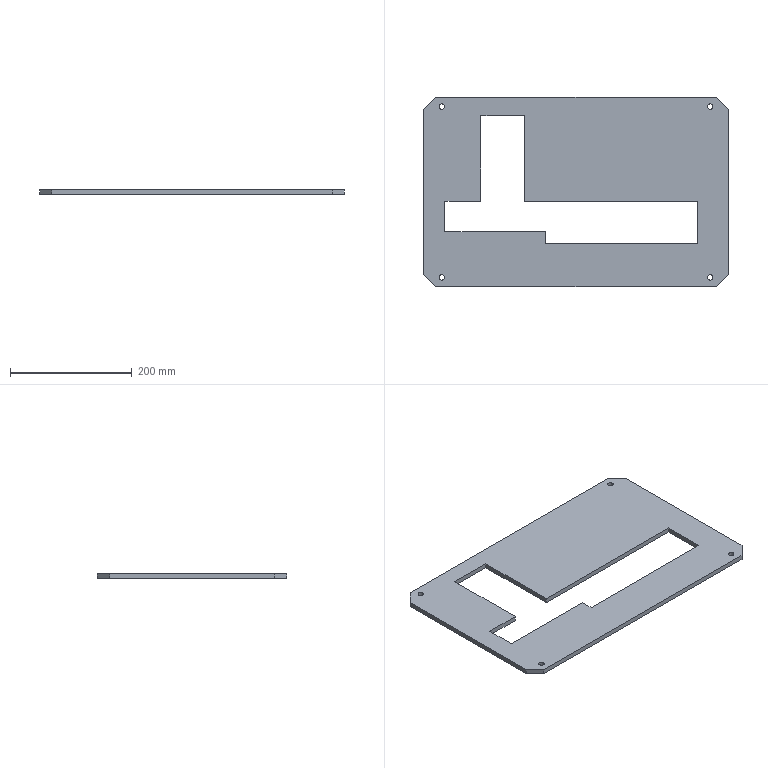Component | SolidWorks | FixedPlateA-1 | 1 solid | 28 faces | box 500 x 310 x 8 mm | volume 944924 mm3 | plane 20 | cylinder 8 | commonest cylinder face diameters 9 x8
STEP:
#1=COLOUR_RGB('',0.7922,0.8196,0.9333);
#2=FILL_AREA_STYLE_COLOUR('',#1);
#3=FILL_AREA_STYLE('',(#2));
#4=SURFACE_STYLE_FILL_AREA(#3);
#5=SURFACE_SIDE_STYLE('',(#4));
#6=SURFACE_STYLE_USAGE(.BOTH.,#5);
#7=PRESENTATION_STYLE_ASSIGNMENT((#6));
#8=CARTESIAN_POINT('',(-8.484,5.512,5.827));
#9=VERTEX_POINT('',#8);
#10=CARTESIAN_POINT('',(-8.839,5.512,5.827));
#11=VERTEX_POINT('',#10);
#12=CARTESIAN_POINT('',(-8.661,5.512,5.827));
#13=DIRECTION('',(0.,0.,-1.));
#14=DIRECTION('',(1.,0.,0.));
#15=AXIS2_PLACEMENT_3D('',#12,#13,#14);
#16=CIRCLE('',#15,0.1772);
#17=EDGE_CURVE('',#9,#11,#16,.T.);
#18=ORIENTED_EDGE('',*,*,#17,.T.);
#19=CARTESIAN_POINT('',(-8.839,5.512,6.142));
#20=VERTEX_POINT('',#19);
#21=CARTESIAN_POINT('',(-8.839,5.512,5.827));
#22=DIRECTION('',(0.,0.,1.));
#23=VECTOR('',#22,39.37);
#24=LINE('',#21,#23);
#25=EDGE_CURVE('',#11,#20,#24,.T.);
#26=ORIENTED_EDGE('',*,*,#25,.T.);
#27=CARTESIAN_POINT('',(-8.484,5.512,6.142));
#28=VERTEX_POINT('',#27);
#29=CARTESIAN_POINT('',(-8.661,5.512,6.142));
#30=DIRECTION('',(0.,0.,1.));
#31=DIRECTION('',(1.,0.,0.));
#32=AXIS2_PLACEMENT_3D('',#29,#30,#31);
#33=CIRCLE('',#32,0.1772);
#34=EDGE_CURVE('',#20,#28,#33,.T.);
#35=ORIENTED_EDGE('',*,*,#34,.T.);
#36=CARTESIAN_POINT('',(-8.484,5.512,5.827));
#37=DIRECTION('',(0.,0.,1.));
#38=VECTOR('',#37,39.37);
#39=LINE('',#36,#38);
#40=EDGE_CURVE('',#9,#28,#39,.T.);
#41=ORIENTED_EDGE('',*,*,#40,.F.);
#42=EDGE_LOOP('',(#18,#26,#35,#41));
#43=FACE_OUTER_BOUND('',#42,.T.);
#44=CARTESIAN_POINT('',(-8.661,5.512,5.827));
#45=DIRECTION('',(0.,0.,1.));
#46=DIRECTION('',(1.,0.,0.));
#47=AXIS2_PLACEMENT_3D('',#44,#45,#46);
#48=CYLINDRICAL_SURFACE('',#47,0.1772);
#49=ADVANCED_FACE('',(#43),#48,.F.);
#50=CARTESIAN_POINT('',(-8.484,-5.512,5.827));
#51=VERTEX_POINT('',#50);
#52=CARTESIAN_POINT('',(-8.839,-5.512,5.827));
#53=VERTEX_POINT('',#52);
#54=CARTESIAN_POINT('',(-8.661,-5.512,5.827));
#55=DIRECTION('',(0.,0.,-1.));
#56=DIRECTION('',(1.,0.,0.));
#57=AXIS2_PLACEMENT_3D('',#54,#55,#56);
#58=CIRCLE('',#57,0.1772);
#59=EDGE_CURVE('',#51,#53,#58,.T.);
#60=ORIENTED_EDGE('',*,*,#59,.T.);
#61=CARTESIAN_POINT('',(-8.839,-5.512,6.142));
#62=VERTEX_POINT('',#61);
#63=CARTESIAN_POINT('',(-8.839,-5.512,5.827));
#64=DIRECTION('',(0.,0.,1.));
#65=VECTOR('',#64,39.37);
#66=LINE('',#63,#65);
#67=EDGE_CURVE('',#53,#62,#66,.T.);
#68=ORIENTED_EDGE('',*,*,#67,.T.);
#69=CARTESIAN_POINT('',(-8.484,-5.512,6.142));
#70=VERTEX_POINT('',#69);
#71=CARTESIAN_POINT('',(-8.661,-5.512,6.142));
#72=DIRECTION('',(0.,0.,1.));
#73=DIRECTION('',(1.,0.,0.));
#74=AXIS2_PLACEMENT_3D('',#71,#72,#73);
#75=CIRCLE('',#74,0.1772);
#76=EDGE_CURVE('',#62,#70,#75,.T.);
#77=ORIENTED_EDGE('',*,*,#76,.T.);
#78=CARTESIAN_POINT('',(-8.484,-5.512,5.827));
#79=DIRECTION('',(0.,0.,1.));
#80=VECTOR('',#79,39.37);
#81=LINE('',#78,#80);
#82=EDGE_CURVE('',#51,#70,#81,.T.);
#83=ORIENTED_EDGE('',*,*,#82,.F.);
#84=EDGE_LOOP('',(#60,#68,#77,#83));
#85=FACE_OUTER_BOUND('',#84,.T.);
#86=CARTESIAN_POINT('',(-8.661,-5.512,5.827));
#87=DIRECTION('',(0.,0.,1.));
#88=DIRECTION('',(1.,0.,0.));
#89=AXIS2_PLACEMENT_3D('',#86,#87,#88);
#90=CYLINDRICAL_SURFACE('',#89,0.1772);
#91=ADVANCED_FACE('',(#85),#90,.F.);
#92=CARTESIAN_POINT('',(8.839,-5.512,5.827));
#93=VERTEX_POINT('',#92);
#94=CARTESIAN_POINT('',(8.484,-5.512,5.827));
#95=VERTEX_POINT('',#94);
#96=CARTESIAN_POINT('',(8.661,-5.512,5.827));
#97=DIRECTION('',(0.,0.,-1.));
#98=DIRECTION('',(1.,0.,0.));
#99=AXIS2_PLACEMENT_3D('',#96,#97,#98);
#100=CIRCLE('',#99,0.1772);
#101=EDGE_CURVE('',#93,#95,#100,.T.);
#102=ORIENTED_EDGE('',*,*,#101,.T.);
#103=CARTESIAN_POINT('',(8.484,-5.512,6.142));
#104=VERTEX_POINT('',#103);
#105=CARTESIAN_POINT('',(8.484,-5.512,5.827));
#106=DIRECTION('',(0.,0.,1.));
#107=VECTOR('',#106,39.37);
#108=LINE('',#105,#107);
#109=EDGE_CURVE('',#95,#104,#108,.T.);
#110=ORIENTED_EDGE('',*,*,#109,.T.);
#111=CARTESIAN_POINT('',(8.839,-5.512,6.142));
#112=VERTEX_POINT('',#111);
#113=CARTESIAN_POINT('',(8.661,-5.512,6.142));
#114=DIRECTION('',(0.,0.,1.));
#115=DIRECTION('',(1.,0.,0.));
#116=AXIS2_PLACEMENT_3D('',#113,#114,#115);
#117=CIRCLE('',#116,0.1772);
#118=EDGE_CURVE('',#104,#112,#117,.T.);
#119=ORIENTED_EDGE('',*,*,#118,.T.);
#120=CARTESIAN_POINT('',(8.839,-5.512,5.827));
#121=DIRECTION('',(0.,0.,1.));
#122=VECTOR('',#121,39.37);
#123=LINE('',#120,#122);
#124=EDGE_CURVE('',#93,#112,#123,.T.);
#125=ORIENTED_EDGE('',*,*,#124,.F.);
#126=EDGE_LOOP('',(#102,#110,#119,#125));
#127=FACE_OUTER_BOUND('',#126,.T.);
#128=CARTESIAN_POINT('',(8.661,-5.512,5.827));
#129=DIRECTION('',(0.,0.,1.));
#130=DIRECTION('',(1.,0.,0.));
#131=AXIS2_PLACEMENT_3D('',#128,#129,#130);
#132=CYLINDRICAL_SURFACE('',#131,0.1772);
#133=ADVANCED_FACE('',(#127),#132,.F.);
#134=CARTESIAN_POINT('',(8.839,5.512,5.827));
#135=VERTEX_POINT('',#134);
#136=CARTESIAN_POINT('',(8.484,5.512,5.827));
#137=VERTEX_POINT('',#136);
#138=CARTESIAN_POINT('',(8.661,5.512,5.827));
#139=DIRECTION('',(0.,0.,-1.));
#140=DIRECTION('',(1.,0.,0.));
#141=AXIS2_PLACEMENT_3D('',#138,#139,#140);
#142=CIRCLE('',#141,0.1772);
#143=EDGE_CURVE('',#135,#137,#142,.T.);
#144=ORIENTED_EDGE('',*,*,#143,.T.);
#145=CARTESIAN_POINT('',(8.484,5.512,6.142));
#146=VERTEX_POINT('',#145);
#147=CARTESIAN_POINT('',(8.484,5.512,5.827));
#148=DIRECTION('',(0.,0.,1.));
#149=VECTOR('',#148,39.37);
#150=LINE('',#147,#149);
#151=EDGE_CURVE('',#137,#146,#150,.T.);
#152=ORIENTED_EDGE('',*,*,#151,.T.);
#153=CARTESIAN_POINT('',(8.839,5.512,6.142));
#154=VERTEX_POINT('',#153);
#155=CARTESIAN_POINT('',(8.661,5.512,6.142));
#156=DIRECTION('',(0.,0.,1.));
#157=DIRECTION('',(1.,0.,0.));
#158=AXIS2_PLACEMENT_3D('',#155,#156,#157);
#159=CIRCLE('',#158,0.1772);
#160=EDGE_CURVE('',#146,#154,#159,.T.);
#161=ORIENTED_EDGE('',*,*,#160,.T.);
#162=CARTESIAN_POINT('',(8.839,5.512,5.827));
#163=DIRECTION('',(0.,0.,1.));
#164=VECTOR('',#163,39.37);
#165=LINE('',#162,#164);
#166=EDGE_CURVE('',#135,#154,#165,.T.);
#167=ORIENTED_EDGE('',*,*,#166,.F.);
#168=EDGE_LOOP('',(#144,#152,#161,#167));
#169=FACE_OUTER_BOUND('',#168,.T.);
#170=CARTESIAN_POINT('',(8.661,5.512,5.827));
#171=DIRECTION('',(0.,0.,1.));
#172=DIRECTION('',(1.,0.,0.));
#173=AXIS2_PLACEMENT_3D('',#170,#171,#172);
#174=CYLINDRICAL_SURFACE('',#173,0.1772);
#175=ADVANCED_FACE('',(#169),#174,.F.);
#176=CARTESIAN_POINT('',(-1.969,-3.346,6.142));
#177=VERTEX_POINT('',#176);
#178=CARTESIAN_POINT('',(7.874,-3.346,6.142));
#179=VERTEX_POINT('',#178);
#180=CARTESIAN_POINT('',(-1.969,-3.346,6.142));
#181=DIRECTION('',(1.,0.,0.));
#182=VECTOR('',#181,39.37);
#183=LINE('',#180,#182);
#184=EDGE_CURVE('',#177,#179,#183,.T.);
#185=ORIENTED_EDGE('',*,*,#184,.T.);
#186=CARTESIAN_POINT('',(7.874,-3.346,5.827));
#187=VERTEX_POINT('',#186);
#188=CARTESIAN_POINT('',(7.874,-3.346,5.827));
#189=DIRECTION('',(0.,0.,1.));
#190=VECTOR('',#189,39.37);
#191=LINE('',#188,#190);
#192=EDGE_CURVE('',#187,#179,#191,.T.);
#193=ORIENTED_EDGE('',*,*,#192,.F.);
#194=CARTESIAN_POINT('',(-1.969,-3.346,5.827));
#195=VERTEX_POINT('',#194);
#196=CARTESIAN_POINT('',(-1.969,-3.346,5.827));
#197=DIRECTION('',(1.,0.,0.));
#198=VECTOR('',#197,39.37);
#199=LINE('',#196,#198);
#200=EDGE_CURVE('',#195,#187,#199,.T.);
#201=ORIENTED_EDGE('',*,*,#200,.F.);
#202=CARTESIAN_POINT('',(-1.969,-3.346,5.827));
#203=DIRECTION('',(0.,0.,1.));
#204=VECTOR('',#203,39.37);
#205=LINE('',#202,#204);
#206=EDGE_CURVE('',#195,#177,#205,.T.);
#207=ORIENTED_EDGE('',*,*,#206,.T.);
#208=EDGE_LOOP('',(#185,#193,#201,#207));
#209=FACE_OUTER_BOUND('',#208,.T.);
#210=CARTESIAN_POINT('',(-1.969,-3.346,5.827));
#211=DIRECTION('',(0.,-1.,0.));
#212=DIRECTION('',(0.,0.,-1.));
#213=AXIS2_PLACEMENT_3D('',#210,#211,#212);
#214=PLANE('',#213);
#215=ADVANCED_FACE('',(#209),#214,.F.);
#216=CARTESIAN_POINT('',(-1.969,-2.559,6.142));
#217=VERTEX_POINT('',#216);
#218=CARTESIAN_POINT('',(-1.969,-2.559,6.142));
#219=DIRECTION('',(0.,-1.,0.));
#220=VECTOR('',#219,39.37);
#221=LINE('',#218,#220);
#222=EDGE_CURVE('',#217,#177,#221,.T.);
#223=ORIENTED_EDGE('',*,*,#222,.T.);
#224=ORIENTED_EDGE('',*,*,#206,.F.);
#225=CARTESIAN_POINT('',(-1.969,-2.559,5.827));
#226=VERTEX_POINT('',#225);
#227=CARTESIAN_POINT('',(-1.969,-2.559,5.827));
#228=DIRECTION('',(0.,-1.,0.));
#229=VECTOR('',#228,39.37);
#230=LINE('',#227,#229);
#231=EDGE_CURVE('',#226,#195,#230,.T.);
#232=ORIENTED_EDGE('',*,*,#231,.F.);
#233=CARTESIAN_POINT('',(-1.969,-2.559,5.827));
#234=DIRECTION('',(0.,0.,1.));
#235=VECTOR('',#234,39.37);
#236=LINE('',#233,#235);
#237=EDGE_CURVE('',#226,#217,#236,.T.);
#238=ORIENTED_EDGE('',*,*,#237,.T.);
#239=EDGE_LOOP('',(#223,#224,#232,#238));
#240=FACE_OUTER_BOUND('',#239,.T.);
#241=CARTESIAN_POINT('',(-1.969,-2.559,5.827));
#242=DIRECTION('',(-1.,0.,0.));
#243=DIRECTION('',(0.,0.,1.));
#244=AXIS2_PLACEMENT_3D('',#241,#242,#243);
#245=PLANE('',#244);
#246=ADVANCED_FACE('',(#240),#245,.F.);
#247=CARTESIAN_POINT('',(-3.307,4.921,6.142));
#248=VERTEX_POINT('',#247);
#249=CARTESIAN_POINT('',(-6.142,4.921,6.142));
#250=VERTEX_POINT('',#249);
#251=CARTESIAN_POINT('',(-3.307,4.921,6.142));
#252=DIRECTION('',(-1.,-0.,0.));
#253=VECTOR('',#252,39.37);
#254=LINE('',#251,#253);
#255=EDGE_CURVE('',#248,#250,#254,.T.);
#256=ORIENTED_EDGE('',*,*,#255,.T.);
#257=CARTESIAN_POINT('',(-6.142,4.921,5.827));
#258=VERTEX_POINT('',#257);
#259=CARTESIAN_POINT('',(-6.142,4.921,5.827));
#260=DIRECTION('',(0.,0.,1.));
#261=VECTOR('',#260,39.37);
#262=LINE('',#259,#261);
#263=EDGE_CURVE('',#258,#250,#262,.T.);
#264=ORIENTED_EDGE('',*,*,#263,.F.);
#265=CARTESIAN_POINT('',(-3.307,4.921,5.827));
#266=VERTEX_POINT('',#265);
#267=CARTESIAN_POINT('',(-3.307,4.921,5.827));
#268=DIRECTION('',(-1.,-0.,0.));
#269=VECTOR('',#268,39.37);
#270=LINE('',#267,#269);
#271=EDGE_CURVE('',#266,#258,#270,.T.);
#272=ORIENTED_EDGE('',*,*,#271,.F.);
#273=CARTESIAN_POINT('',(-3.307,4.921,5.827));
#274=DIRECTION('',(0.,0.,1.));
#275=VECTOR('',#274,39.37);
#276=LINE('',#273,#275);
#277=EDGE_CURVE('',#266,#248,#276,.T.);
#278=ORIENTED_EDGE('',*,*,#277,.T.);
#279=EDGE_LOOP('',(#256,#264,#272,#278));
#280=FACE_OUTER_BOUND('',#279,.T.);
#281=CARTESIAN_POINT('',(-3.307,4.921,5.827));
#282=DIRECTION('',(-0.,1.,0.));
#283=DIRECTION('',(1.,0.,0.));
#284=AXIS2_PLACEMENT_3D('',#281,#282,#283);
#285=PLANE('',#284);
#286=ADVANCED_FACE('',(#280),#285,.F.);
#287=CARTESIAN_POINT('',(-6.142,-0.5906,6.142));
#288=VERTEX_POINT('',#287);
#289=CARTESIAN_POINT('',(-6.142,4.921,6.142));
#290=DIRECTION('',(-0.,-1.,0.));
#291=VECTOR('',#290,39.37);
#292=LINE('',#289,#291);
#293=EDGE_CURVE('',#250,#288,#292,.T.);
#294=ORIENTED_EDGE('',*,*,#293,.T.);
#295=CARTESIAN_POINT('',(-6.142,-0.5906,5.827));
#296=VERTEX_POINT('',#295);
#297=CARTESIAN_POINT('',(-6.142,-0.5906,5.827));
#298=DIRECTION('',(0.,0.,1.));
#299=VECTOR('',#298,39.37);
#300=LINE('',#297,#299);
#301=EDGE_CURVE('',#296,#288,#300,.T.);
#302=ORIENTED_EDGE('',*,*,#301,.F.);
#303=CARTESIAN_POINT('',(-6.142,4.921,5.827));
#304=DIRECTION('',(-0.,-1.,0.));
#305=VECTOR('',#304,39.37);
#306=LINE('',#303,#305);
#307=EDGE_CURVE('',#258,#296,#306,.T.);
#308=ORIENTED_EDGE('',*,*,#307,.F.);
#309=ORIENTED_EDGE('',*,*,#263,.T.);
#310=EDGE_LOOP('',(#294,#302,#308,#309));
#311=FACE_OUTER_BOUND('',#310,.T.);
#312=CARTESIAN_POINT('',(-6.142,4.921,5.827));
#313=DIRECTION('',(-1.,0.,0.));
#314=DIRECTION('',(0.,0.,1.));
#315=AXIS2_PLACEMENT_3D('',#312,#313,#314);
#316=PLANE('',#315);
#317=ADVANCED_FACE('',(#311),#316,.F.);
#318=CARTESIAN_POINT('',(-3.307,-0.5906,6.142));
#319=VERTEX_POINT('',#318);
#320=CARTESIAN_POINT('',(-3.307,4.921,6.142));
#321=DIRECTION('',(-0.,1.,0.));
#322=VECTOR('',#321,39.37);
#323=LINE('',#320,#322);
#324=EDGE_CURVE('',#319,#248,#323,.T.);
#325=ORIENTED_EDGE('',*,*,#324,.T.);
#326=ORIENTED_EDGE('',*,*,#277,.F.);
#327=CARTESIAN_POINT('',(-3.307,-0.5906,5.827));
#328=VERTEX_POINT('',#327);
#329=CARTESIAN_POINT('',(-3.307,4.921,5.827));
#330=DIRECTION('',(-0.,1.,0.));
#331=VECTOR('',#330,39.37);
#332=LINE('',#329,#331);
#333=EDGE_CURVE('',#328,#266,#332,.T.);
#334=ORIENTED_EDGE('',*,*,#333,.F.);
#335=CARTESIAN_POINT('',(-3.307,-0.5906,5.827));
#336=DIRECTION('',(0.,0.,1.));
#337=VECTOR('',#336,39.37);
#338=LINE('',#335,#337);
#339=EDGE_CURVE('',#328,#319,#338,.T.);
#340=ORIENTED_EDGE('',*,*,#339,.T.);
#341=EDGE_LOOP('',(#325,#326,#334,#340));
#342=FACE_OUTER_BOUND('',#341,.T.);
#343=CARTESIAN_POINT('',(-3.307,4.921,5.827));
#344=DIRECTION('',(1.,0.,0.));
#345=DIRECTION('',(-0.,1.,0.));
#346=AXIS2_PLACEMENT_3D('',#343,#344,#345);
#347=PLANE('',#346);
#348=ADVANCED_FACE('',(#342),#347,.F.);
#349=CARTESIAN_POINT('',(-8.465,-2.559,6.142));
#350=VERTEX_POINT('',#349);
#351=CARTESIAN_POINT('',(7.874,-2.559,6.142));
#352=DIRECTION('',(1.,0.,0.));
#353=VECTOR('',#352,39.37);
#354=LINE('',#351,#353);
#355=EDGE_CURVE('',#350,#217,#354,.T.);
#356=ORIENTED_EDGE('',*,*,#355,.T.);
#357=ORIENTED_EDGE('',*,*,#237,.F.);
#358=CARTESIAN_POINT('',(-8.465,-2.559,5.827));
#359=VERTEX_POINT('',#358);
#360=CARTESIAN_POINT('',(7.874,-2.559,5.827));
#361=DIRECTION('',(1.,0.,0.));
#362=VECTOR('',#361,39.37);
#363=LINE('',#360,#362);
#364=EDGE_CURVE('',#359,#226,#363,.T.);
#365=ORIENTED_EDGE('',*,*,#364,.F.);
#366=CARTESIAN_POINT('',(-8.465,-2.559,5.827));
#367=DIRECTION('',(0.,0.,1.));
#368=VECTOR('',#367,39.37);
#369=LINE('',#366,#368);
#370=EDGE_CURVE('',#359,#350,#369,.T.);
#371=ORIENTED_EDGE('',*,*,#370,.T.);
#372=EDGE_LOOP('',(#356,#357,#365,#371));
#373=FACE_OUTER_BOUND('',#372,.T.);
#374=CARTESIAN_POINT('',(7.874,-2.559,5.827));
#375=DIRECTION('',(0.,-1.,0.));
#376=DIRECTION('',(0.,0.,-1.));
#377=AXIS2_PLACEMENT_3D('',#374,#375,#376);
#378=PLANE('',#377);
#379=ADVANCED_FACE('',(#373),#378,.F.);
#380=CARTESIAN_POINT('',(7.874,-0.5906,6.142));
#381=VERTEX_POINT('',#380);
#382=CARTESIAN_POINT('',(7.874,-0.5906,6.142));
#383=DIRECTION('',(0.,1.,0.));
#384=VECTOR('',#383,39.37);
#385=LINE('',#382,#384);
#386=EDGE_CURVE('',#179,#381,#385,.T.);
#387=ORIENTED_EDGE('',*,*,#386,.T.);
#388=CARTESIAN_POINT('',(7.874,-0.5906,5.827));
#389=VERTEX_POINT('',#388);
#390=CARTESIAN_POINT('',(7.874,-0.5906,5.827));
#391=DIRECTION('',(0.,0.,1.));
#392=VECTOR('',#391,39.37);
#393=LINE('',#390,#392);
#394=EDGE_CURVE('',#389,#381,#393,.T.);
#395=ORIENTED_EDGE('',*,*,#394,.F.);
#396=CARTESIAN_POINT('',(7.874,-0.5906,5.827));
#397=DIRECTION('',(0.,1.,0.));
#398=VECTOR('',#397,39.37);
#399=LINE('',#396,#398);
#400=EDGE_CURVE('',#187,#389,#399,.T.);
#401=ORIENTED_EDGE('',*,*,#400,.F.);
#402=ORIENTED_EDGE('',*,*,#192,.T.);
#403=EDGE_LOOP('',(#387,#395,#401,#402));
#404=FACE_OUTER_BOUND('',#403,.T.);
#405=CARTESIAN_POINT('',(7.874,-0.5906,5.827));
#406=DIRECTION('',(1.,0.,0.));
#407=DIRECTION('',(0.,1.,0.));
#408=AXIS2_PLACEMENT_3D('',#405,#406,#407);
#409=PLANE('',#408);
#410=ADVANCED_FACE('',(#404),#409,.F.);
#411=CARTESIAN_POINT('',(-8.465,-0.5906,5.827));
#412=VERTEX_POINT('',#411);
#413=CARTESIAN_POINT('',(-8.465,-0.5906,5.827));
#414=DIRECTION('',(-1.,0.,0.));
#415=VECTOR('',#414,39.37);
#416=LINE('',#413,#415);
#417=EDGE_CURVE('',#296,#412,#416,.T.);
#418=ORIENTED_EDGE('',*,*,#417,.F.);
#419=ORIENTED_EDGE('',*,*,#301,.T.);
#420=CARTESIAN_POINT('',(-8.465,-0.5906,6.142));
#421=VERTEX_POINT('',#420);
#422=CARTESIAN_POINT('',(-8.465,-0.5906,6.142));
#423=DIRECTION('',(-1.,0.,0.));
#424=VECTOR('',#423,39.37);
#425=LINE('',#422,#424);
#426=EDGE_CURVE('',#288,#421,#425,.T.);
#427=ORIENTED_EDGE('',*,*,#426,.T.);
#428=CARTESIAN_POINT('',(-8.465,-0.5906,5.827));
#429=DIRECTION('',(0.,0.,1.));
#430=VECTOR('',#429,39.37);
#431=LINE('',#428,#430);
#432=EDGE_CURVE('',#412,#421,#431,.T.);
#433=ORIENTED_EDGE('',*,*,#432,.F.);
#434=EDGE_LOOP('',(#418,#419,#427,#433));
#435=FACE_OUTER_BOUND('',#434,.T.);
#436=CARTESIAN_POINT('',(-8.465,-0.5906,5.827));
#437=DIRECTION('',(0.,1.,0.));
#438=DIRECTION('',(1.,0.,0.));
#439=AXIS2_PLACEMENT_3D('',#436,#437,#438);
#440=PLANE('',#439);
#441=ADVANCED_FACE('',(#435),#440,.F.);
#442=CARTESIAN_POINT('',(-8.465,-2.559,6.142));
#443=DIRECTION('',(0.,-1.,0.));
#444=VECTOR('',#443,39.37);
#445=LINE('',#442,#444);
#446=EDGE_CURVE('',#421,#350,#445,.T.);
#447=ORIENTED_EDGE('',*,*,#446,.T.);
#448=ORIENTED_EDGE('',*,*,#370,.F.);
#449=CARTESIAN_POINT('',(-8.465,-2.559,5.827));
#450=DIRECTION('',(0.,-1.,0.));
#451=VECTOR('',#450,39.37);
#452=LINE('',#449,#451);
#453=EDGE_CURVE('',#412,#359,#452,.T.);
#454=ORIENTED_EDGE('',*,*,#453,.F.);
#455=ORIENTED_EDGE('',*,*,#432,.T.);
#456=EDGE_LOOP('',(#447,#448,#454,#455));
#457=FACE_OUTER_BOUND('',#456,.T.);
#458=CARTESIAN_POINT('',(-8.465,-2.559,5.827));
#459=DIRECTION('',(-1.,0.,0.));
#460=DIRECTION('',(0.,0.,1.));
#461=AXIS2_PLACEMENT_3D('',#458,#459,#460);
#462=PLANE('',#461);
#463=ADVANCED_FACE('',(#457),#462,.F.);
#464=CARTESIAN_POINT('',(9.055,-6.102,6.142));
#465=VERTEX_POINT('',#464);
#466=CARTESIAN_POINT('',(9.843,-5.315,6.142));
#467=VERTEX_POINT('',#466);
#468=CARTESIAN_POINT('',(7.579,-7.579,6.142));
#469=DIRECTION('',(0.7071,0.7071,0.));
#470=VECTOR('',#469,39.37);
#471=LINE('',#468,#470);
#472=EDGE_CURVE('',#465,#467,#471,.T.);
#473=ORIENTED_EDGE('',*,*,#472,.F.);
#474=CARTESIAN_POINT('',(9.055,-6.102,5.827));
#475=VERTEX_POINT('',#474);
#476=CARTESIAN_POINT('',(9.055,-6.102,6.142));
#477=DIRECTION('',(0.,0.,1.));
#478=VECTOR('',#477,39.37);
#479=LINE('',#476,#478);
#480=EDGE_CURVE('',#475,#465,#479,.T.);
#481=ORIENTED_EDGE('',*,*,#480,.F.);
#482=CARTESIAN_POINT('',(9.843,-5.315,5.827));
#483=VERTEX_POINT('',#482);
#484=CARTESIAN_POINT('',(9.843,-5.315,5.827));
#485=DIRECTION('',(-0.7071,-0.7071,0.));
#486=VECTOR('',#485,39.37);
#487=LINE('',#484,#486);
#488=EDGE_CURVE('',#483,#475,#487,.T.);
#489=ORIENTED_EDGE('',*,*,#488,.F.);
#490=CARTESIAN_POINT('',(9.843,-5.315,6.142));
#491=DIRECTION('',(0.,0.,-1.));
#492=VECTOR('',#491,39.37);
#493=LINE('',#490,#492);
#494=EDGE_CURVE('',#467,#483,#493,.T.);
#495=ORIENTED_EDGE('',*,*,#494,.F.);
#496=EDGE_LOOP('',(#473,#481,#489,#495));
#497=FACE_OUTER_BOUND('',#496,.T.);
#498=CARTESIAN_POINT('',(9.843,-5.315,6.142));
#499=DIRECTION('',(-0.7071,0.7071,0.));
#500=DIRECTION('',(0.,0.,1.));
#501=AXIS2_PLACEMENT_3D('',#498,#499,#500);
#502=PLANE('',#501);
#503=ADVANCED_FACE('',(#497),#502,.F.);
#504=CARTESIAN_POINT('',(-9.843,-5.315,6.142));
#505=VERTEX_POINT('',#504);
#506=CARTESIAN_POINT('',(-9.055,-6.102,6.142));
#507=VERTEX_POINT('',#506);
#508=CARTESIAN_POINT('',(-7.579,-7.579,6.142));
#509=DIRECTION('',(0.7071,-0.7071,0.));
#510=VECTOR('',#509,39.37);
#511=LINE('',#508,#510);
#512=EDGE_CURVE('',#505,#507,#511,.T.);
#513=ORIENTED_EDGE('',*,*,#512,.F.);
#514=CARTESIAN_POINT('',(-9.843,-5.315,5.827));
#515=VERTEX_POINT('',#514);
#516=CARTESIAN_POINT('',(-9.843,-5.315,6.142));
#517=DIRECTION('',(0.,0.,1.));
#518=VECTOR('',#517,39.37);
#519=LINE('',#516,#518);
#520=EDGE_CURVE('',#515,#505,#519,.T.);
#521=ORIENTED_EDGE('',*,*,#520,.F.);
#522=CARTESIAN_POINT('',(-9.055,-6.102,5.827));
#523=VERTEX_POINT('',#522);
#524=CARTESIAN_POINT('',(-9.055,-6.102,5.827));
#525=DIRECTION('',(-0.7071,0.7071,0.));
#526=VECTOR('',#525,39.37);
#527=LINE('',#524,#526);
#528=EDGE_CURVE('',#523,#515,#527,.T.);
#529=ORIENTED_EDGE('',*,*,#528,.F.);
#530=CARTESIAN_POINT('',(-9.055,-6.102,6.142));
#531=DIRECTION('',(0.,0.,-1.));
#532=VECTOR('',#531,39.37);
#533=LINE('',#530,#532);
#534=EDGE_CURVE('',#507,#523,#533,.T.);
#535=ORIENTED_EDGE('',*,*,#534,.F.);
#536=EDGE_LOOP('',(#513,#521,#529,#535));
#537=FACE_OUTER_BOUND('',#536,.T.);
#538=CARTESIAN_POINT('',(-9.055,-6.102,6.142));
#539=DIRECTION('',(0.7071,0.7071,0.));
#540=DIRECTION('',(0.,0.,-1.));
#541=AXIS2_PLACEMENT_3D('',#538,#539,#540);
#542=PLANE('',#541);
#543=ADVANCED_FACE('',(#537),#542,.F.);
#544=CARTESIAN_POINT('',(-9.055,6.102,6.142));
#545=VERTEX_POINT('',#544);
#546=CARTESIAN_POINT('',(-9.843,5.315,6.142));
#547=VERTEX_POINT('',#546);
#548=CARTESIAN_POINT('',(-7.579,7.579,6.142));
#549=DIRECTION('',(-0.7071,-0.7071,0.));
#550=VECTOR('',#549,39.37);
#551=LINE('',#548,#550);
#552=EDGE_CURVE('',#545,#547,#551,.T.);
#553=ORIENTED_EDGE('',*,*,#552,.F.);
#554=CARTESIAN_POINT('',(-9.055,6.102,5.827));
#555=VERTEX_POINT('',#554);
#556=CARTESIAN_POINT('',(-9.055,6.102,6.142));
#557=DIRECTION('',(0.,0.,1.));
#558=VECTOR('',#557,39.37);
#559=LINE('',#556,#558);
#560=EDGE_CURVE('',#555,#545,#559,.T.);
#561=ORIENTED_EDGE('',*,*,#560,.F.);
#562=CARTESIAN_POINT('',(-9.843,5.315,5.827));
#563=VERTEX_POINT('',#562);
#564=CARTESIAN_POINT('',(-9.843,5.315,5.827));
#565=DIRECTION('',(0.7071,0.7071,0.));
#566=VECTOR('',#565,39.37);
#567=LINE('',#564,#566);
#568=EDGE_CURVE('',#563,#555,#567,.T.);
#569=ORIENTED_EDGE('',*,*,#568,.F.);
#570=CARTESIAN_POINT('',(-9.843,5.315,6.142));
#571=DIRECTION('',(0.,0.,-1.));
#572=VECTOR('',#571,39.37);
#573=LINE('',#570,#572);
#574=EDGE_CURVE('',#547,#563,#573,.T.);
#575=ORIENTED_EDGE('',*,*,#574,.F.);
#576=EDGE_LOOP('',(#553,#561,#569,#575));
#577=FACE_OUTER_BOUND('',#576,.T.);
#578=CARTESIAN_POINT('',(-9.843,5.315,6.142));
#579=DIRECTION('',(0.7071,-0.7071,0.));
#580=DIRECTION('',(0.,0.,-1.));
#581=AXIS2_PLACEMENT_3D('',#578,#579,#580);
#582=PLANE('',#581);
#583=ADVANCED_FACE('',(#577),#582,.F.);
#584=CARTESIAN_POINT('',(9.843,5.315,6.142));
#585=VERTEX_POINT('',#584);
#586=CARTESIAN_POINT('',(9.055,6.102,6.142));
#587=VERTEX_POINT('',#586);
#588=CARTESIAN_POINT('',(7.579,7.579,6.142));
#589=DIRECTION('',(-0.7071,0.7071,0.));
#590=VECTOR('',#589,39.37);
#591=LINE('',#588,#590);
#592=EDGE_CURVE('',#585,#587,#591,.T.);
#593=ORIENTED_EDGE('',*,*,#592,.F.);
#594=CARTESIAN_POINT('',(9.843,5.315,5.827));
#595=VERTEX_POINT('',#594);
#596=CARTESIAN_POINT('',(9.843,5.315,6.142));
#597=DIRECTION('',(0.,0.,1.));
#598=VECTOR('',#597,39.37);
#599=LINE('',#596,#598);
#600=EDGE_CURVE('',#595,#585,#599,.T.);
#601=ORIENTED_EDGE('',*,*,#600,.F.);
#602=CARTESIAN_POINT('',(9.055,6.102,5.827));
#603=VERTEX_POINT('',#602);
#604=CARTESIAN_POINT('',(9.055,6.102,5.827));
#605=DIRECTION('',(0.7071,-0.7071,0.));
#606=VECTOR('',#605,39.37);
#607=LINE('',#604,#606);
#608=EDGE_CURVE('',#603,#595,#607,.T.);
#609=ORIENTED_EDGE('',*,*,#608,.F.);
#610=CARTESIAN_POINT('',(9.055,6.102,6.142));
#611=DIRECTION('',(0.,0.,-1.));
#612=VECTOR('',#611,39.37);
#613=LINE('',#610,#612);
#614=EDGE_CURVE('',#587,#603,#613,.T.);
#615=ORIENTED_EDGE('',*,*,#614,.F.);
#616=EDGE_LOOP('',(#593,#601,#609,#615));
#617=FACE_OUTER_BOUND('',#616,.T.);
#618=CARTESIAN_POINT('',(9.055,6.102,6.142));
#619=DIRECTION('',(-0.7071,-0.7071,0.));
#620=DIRECTION('',(-0.7071,0.7071,0.));
#621=AXIS2_PLACEMENT_3D('',#618,#619,#620);
#622=PLANE('',#621);
#623=ADVANCED_FACE('',(#617),#622,.F.);
#624=ORIENTED_EDGE('',*,*,#17,.F.);
#625=CARTESIAN_POINT('',(-8.661,5.512,5.827));
#626=DIRECTION('',(0.,0.,-1.));
#627=DIRECTION('',(1.,0.,0.));
#628=AXIS2_PLACEMENT_3D('',#625,#626,#627);
#629=CIRCLE('',#628,0.1772);
#630=EDGE_CURVE('',#11,#9,#629,.T.);
#631=ORIENTED_EDGE('',*,*,#630,.F.);
#632=EDGE_LOOP('',(#624,#631));
#633=FACE_BOUND('',#632,.T.);
#634=ORIENTED_EDGE('',*,*,#59,.F.);
#635=CARTESIAN_POINT('',(-8.661,-5.512,5.827));
#636=DIRECTION('',(0.,0.,-1.));
#637=DIRECTION('',(1.,0.,0.));
#638=AXIS2_PLACEMENT_3D('',#635,#636,#637);
#639=CIRCLE('',#638,0.1772);
#640=EDGE_CURVE('',#53,#51,#639,.T.);
#641=ORIENTED_EDGE('',*,*,#640,.F.);
#642=EDGE_LOOP('',(#634,#641));
#643=FACE_BOUND('',#642,.T.);
#644=ORIENTED_EDGE('',*,*,#101,.F.);
#645=CARTESIAN_POINT('',(8.661,-5.512,5.827));
#646=DIRECTION('',(0.,0.,-1.));
#647=DIRECTION('',(1.,0.,0.));
#648=AXIS2_PLACEMENT_3D('',#645,#646,#647);
#649=CIRCLE('',#648,0.1772);
#650=EDGE_CURVE('',#95,#93,#649,.T.);
#651=ORIENTED_EDGE('',*,*,#650,.F.);
#652=EDGE_LOOP('',(#644,#651));
#653=FACE_BOUND('',#652,.T.);
#654=ORIENTED_EDGE('',*,*,#143,.F.);
#655=CARTESIAN_POINT('',(8.661,5.512,5.827));
#656=DIRECTION('',(0.,0.,-1.));
#657=DIRECTION('',(1.,0.,0.));
#658=AXIS2_PLACEMENT_3D('',#655,#656,#657);
#659=CIRCLE('',#658,0.1772);
#660=EDGE_CURVE('',#137,#135,#659,.T.);
#661=ORIENTED_EDGE('',*,*,#660,.F.);
#662=EDGE_LOOP('',(#654,#661));
#663=FACE_BOUND('',#662,.T.);
#664=ORIENTED_EDGE('',*,*,#364,.T.);
#665=ORIENTED_EDGE('',*,*,#231,.T.);
#666=ORIENTED_EDGE('',*,*,#200,.T.);
#667=ORIENTED_EDGE('',*,*,#400,.T.);
#668=CARTESIAN_POINT('',(-8.465,-0.5906,5.827));
#669=DIRECTION('',(-1.,0.,0.));
#670=VECTOR('',#669,39.37);
#671=LINE('',#668,#670);
#672=EDGE_CURVE('',#389,#328,#671,.T.);
#673=ORIENTED_EDGE('',*,*,#672,.T.);
#674=ORIENTED_EDGE('',*,*,#333,.T.);
#675=ORIENTED_EDGE('',*,*,#271,.T.);
#676=ORIENTED_EDGE('',*,*,#307,.T.);
#677=ORIENTED_EDGE('',*,*,#417,.T.);
#678=ORIENTED_EDGE('',*,*,#453,.T.);
#679=EDGE_LOOP('',(#664,#665,#666,#667,#673,#674,#675,#676,#677,#678));
#680=FACE_BOUND('',#679,.T.);
#681=CARTESIAN_POINT('',(-9.843,6.102,5.827));
#682=DIRECTION('',(-1.,0.,0.));
#683=VECTOR('',#682,39.37);
#684=LINE('',#681,#683);
#685=EDGE_CURVE('',#603,#555,#684,.T.);
#686=ORIENTED_EDGE('',*,*,#685,.F.);
#687=ORIENTED_EDGE('',*,*,#608,.T.);
#688=CARTESIAN_POINT('',(9.843,6.102,5.827));
#689=DIRECTION('',(0.,1.,0.));
#690=VECTOR('',#689,39.37);
#691=LINE('',#688,#690);
#692=EDGE_CURVE('',#483,#595,#691,.T.);
#693=ORIENTED_EDGE('',*,*,#692,.F.);
#694=ORIENTED_EDGE('',*,*,#488,.T.);
#695=CARTESIAN_POINT('',(-9.843,-6.102,5.827));
#696=DIRECTION('',(1.,0.,0.));
#697=VECTOR('',#696,39.37);
#698=LINE('',#695,#697);
#699=EDGE_CURVE('',#523,#475,#698,.T.);
#700=ORIENTED_EDGE('',*,*,#699,.F.);
#701=ORIENTED_EDGE('',*,*,#528,.T.);
#702=CARTESIAN_POINT('',(-9.843,6.102,5.827));
#703=DIRECTION('',(0.,-1.,0.));
#704=VECTOR('',#703,39.37);
#705=LINE('',#702,#704);
#706=EDGE_CURVE('',#563,#515,#705,.T.);
#707=ORIENTED_EDGE('',*,*,#706,.F.);
#708=ORIENTED_EDGE('',*,*,#568,.T.);
#709=EDGE_LOOP('',(#686,#687,#693,#694,#700,#701,#707,#708));
#710=FACE_OUTER_BOUND('',#709,.T.);
#711=CARTESIAN_POINT('',(0.,0.,5.827));
#712=DIRECTION('',(0.,0.,1.));
#713=DIRECTION('',(1.,0.,0.));
#714=AXIS2_PLACEMENT_3D('',#711,#712,#713);
#715=PLANE('',#714);
#716=ADVANCED_FACE('',(#633,#643,#653,#663,#680,#710),#715,.F.);
#717=CARTESIAN_POINT('',(-8.661,5.512,6.142));
#718=DIRECTION('',(0.,0.,1.));
#719=DIRECTION('',(1.,0.,0.));
#720=AXIS2_PLACEMENT_3D('',#717,#718,#719);
#721=CIRCLE('',#720,0.1772);
#722=EDGE_CURVE('',#28,#20,#721,.T.);
#723=ORIENTED_EDGE('',*,*,#722,.F.);
#724=ORIENTED_EDGE('',*,*,#34,.F.);
#725=EDGE_LOOP('',(#723,#724));
#726=FACE_BOUND('',#725,.T.);
#727=CARTESIAN_POINT('',(-8.661,-5.512,6.142));
#728=DIRECTION('',(0.,0.,1.));
#729=DIRECTION('',(1.,0.,0.));
#730=AXIS2_PLACEMENT_3D('',#727,#728,#729);
#731=CIRCLE('',#730,0.1772);
#732=EDGE_CURVE('',#70,#62,#731,.T.);
#733=ORIENTED_EDGE('',*,*,#732,.F.);
#734=ORIENTED_EDGE('',*,*,#76,.F.);
#735=EDGE_LOOP('',(#733,#734));
#736=FACE_BOUND('',#735,.T.);
#737=CARTESIAN_POINT('',(8.661,-5.512,6.142));
#738=DIRECTION('',(0.,0.,1.));
#739=DIRECTION('',(1.,0.,0.));
#740=AXIS2_PLACEMENT_3D('',#737,#738,#739);
#741=CIRCLE('',#740,0.1772);
#742=EDGE_CURVE('',#112,#104,#741,.T.);
#743=ORIENTED_EDGE('',*,*,#742,.F.);
#744=ORIENTED_EDGE('',*,*,#118,.F.);
#745=EDGE_LOOP('',(#743,#744));
#746=FACE_BOUND('',#745,.T.);
#747=CARTESIAN_POINT('',(8.661,5.512,6.142));
#748=DIRECTION('',(0.,0.,1.));
#749=DIRECTION('',(1.,0.,0.));
#750=AXIS2_PLACEMENT_3D('',#747,#748,#749);
#751=CIRCLE('',#750,0.1772);
#752=EDGE_CURVE('',#154,#146,#751,.T.);
#753=ORIENTED_EDGE('',*,*,#752,.F.);
#754=ORIENTED_EDGE('',*,*,#160,.F.);
#755=EDGE_LOOP('',(#753,#754));
#756=FACE_BOUND('',#755,.T.);
#757=ORIENTED_EDGE('',*,*,#222,.F.);
#758=ORIENTED_EDGE('',*,*,#355,.F.);
#759=ORIENTED_EDGE('',*,*,#446,.F.);
#760=ORIENTED_EDGE('',*,*,#426,.F.);
#761=ORIENTED_EDGE('',*,*,#293,.F.);
#762=ORIENTED_EDGE('',*,*,#255,.F.);
#763=ORIENTED_EDGE('',*,*,#324,.F.);
#764=CARTESIAN_POINT('',(-8.465,-0.5906,6.142));
#765=DIRECTION('',(-1.,0.,0.));
#766=VECTOR('',#765,39.37);
#767=LINE('',#764,#766);
#768=EDGE_CURVE('',#381,#319,#767,.T.);
#769=ORIENTED_EDGE('',*,*,#768,.F.);
#770=ORIENTED_EDGE('',*,*,#386,.F.);
#771=ORIENTED_EDGE('',*,*,#184,.F.);
#772=EDGE_LOOP('',(#757,#758,#759,#760,#761,#762,#763,#769,#770,#771));
#773=FACE_BOUND('',#772,.T.);
#774=CARTESIAN_POINT('',(9.843,6.102,6.142));
#775=DIRECTION('',(0.,1.,0.));
#776=VECTOR('',#775,39.37);
#777=LINE('',#774,#776);
#778=EDGE_CURVE('',#467,#585,#777,.T.);
#779=ORIENTED_EDGE('',*,*,#778,.T.);
#780=ORIENTED_EDGE('',*,*,#592,.T.);
#781=CARTESIAN_POINT('',(-9.843,6.102,6.142));
#782=DIRECTION('',(-1.,0.,0.));
#783=VECTOR('',#782,39.37);
#784=LINE('',#781,#783);
#785=EDGE_CURVE('',#587,#545,#784,.T.);
#786=ORIENTED_EDGE('',*,*,#785,.T.);
#787=ORIENTED_EDGE('',*,*,#552,.T.);
#788=CARTESIAN_POINT('',(-9.843,6.102,6.142));
#789=DIRECTION('',(0.,-1.,0.));
#790=VECTOR('',#789,39.37);
#791=LINE('',#788,#790);
#792=EDGE_CURVE('',#547,#505,#791,.T.);
#793=ORIENTED_EDGE('',*,*,#792,.T.);
#794=ORIENTED_EDGE('',*,*,#512,.T.);
#795=CARTESIAN_POINT('',(-9.843,-6.102,6.142));
#796=DIRECTION('',(1.,0.,0.));
#797=VECTOR('',#796,39.37);
#798=LINE('',#795,#797);
#799=EDGE_CURVE('',#507,#465,#798,.T.);
#800=ORIENTED_EDGE('',*,*,#799,.T.);
#801=ORIENTED_EDGE('',*,*,#472,.T.);
#802=EDGE_LOOP('',(#779,#780,#786,#787,#793,#794,#800,#801));
#803=FACE_OUTER_BOUND('',#802,.T.);
#804=CARTESIAN_POINT('',(0.,0.,6.142));
#805=DIRECTION('',(0.,0.,1.));
#806=DIRECTION('',(1.,0.,0.));
#807=AXIS2_PLACEMENT_3D('',#804,#805,#806);
#808=PLANE('',#807);
#809=ADVANCED_FACE('',(#726,#736,#746,#756,#773,#803),#808,.T.);
#810=ORIENTED_EDGE('',*,*,#799,.F.);
#811=ORIENTED_EDGE('',*,*,#534,.T.);
#812=ORIENTED_EDGE('',*,*,#699,.T.);
#813=ORIENTED_EDGE('',*,*,#480,.T.);
#814=EDGE_LOOP('',(#810,#811,#812,#813));
#815=FACE_OUTER_BOUND('',#814,.T.);
#816=CARTESIAN_POINT('',(-9.843,-6.102,6.142));
#817=DIRECTION('',(0.,1.,0.));
#818=DIRECTION('',(1.,0.,0.));
#819=AXIS2_PLACEMENT_3D('',#816,#817,#818);
#820=PLANE('',#819);
#821=ADVANCED_FACE('',(#815),#820,.F.);
#822=ORIENTED_EDGE('',*,*,#792,.F.);
#823=ORIENTED_EDGE('',*,*,#574,.T.);
#824=ORIENTED_EDGE('',*,*,#706,.T.);
#825=ORIENTED_EDGE('',*,*,#520,.T.);
#826=EDGE_LOOP('',(#822,#823,#824,#825));
#827=FACE_OUTER_BOUND('',#826,.T.);
#828=CARTESIAN_POINT('',(-9.843,6.102,6.142));
#829=DIRECTION('',(1.,0.,0.));
#830=DIRECTION('',(0.,1.,0.));
#831=AXIS2_PLACEMENT_3D('',#828,#829,#830);
#832=PLANE('',#831);
#833=ADVANCED_FACE('',(#827),#832,.F.);
#834=ORIENTED_EDGE('',*,*,#785,.F.);
#835=ORIENTED_EDGE('',*,*,#614,.T.);
#836=ORIENTED_EDGE('',*,*,#685,.T.);
#837=ORIENTED_EDGE('',*,*,#560,.T.);
#838=EDGE_LOOP('',(#834,#835,#836,#837));
#839=FACE_OUTER_BOUND('',#838,.T.);
#840=CARTESIAN_POINT('',(-9.843,6.102,6.142));
#841=DIRECTION('',(0.,-1.,0.));
#842=DIRECTION('',(0.,0.,-1.));
#843=AXIS2_PLACEMENT_3D('',#840,#841,#842);
#844=PLANE('',#843);
#845=ADVANCED_FACE('',(#839),#844,.F.);
#846=ORIENTED_EDGE('',*,*,#692,.T.);
#847=ORIENTED_EDGE('',*,*,#600,.T.);
#848=ORIENTED_EDGE('',*,*,#778,.F.);
#849=ORIENTED_EDGE('',*,*,#494,.T.);
#850=EDGE_LOOP('',(#846,#847,#848,#849));
#851=FACE_OUTER_BOUND('',#850,.T.);
#852=CARTESIAN_POINT('',(9.843,6.102,6.142));
#853=DIRECTION('',(-1.,0.,0.));
#854=DIRECTION('',(0.,0.,1.));
#855=AXIS2_PLACEMENT_3D('',#852,#853,#854);
#856=PLANE('',#855);
#857=ADVANCED_FACE('',(#851),#856,.F.);
#858=ORIENTED_EDGE('',*,*,#768,.T.);
#859=ORIENTED_EDGE('',*,*,#339,.F.);
#860=ORIENTED_EDGE('',*,*,#672,.F.);
#861=ORIENTED_EDGE('',*,*,#394,.T.);
#862=EDGE_LOOP('',(#858,#859,#860,#861));
#863=FACE_OUTER_BOUND('',#862,.T.);
#864=CARTESIAN_POINT('',(-8.465,-0.5906,5.827));
#865=DIRECTION('',(0.,1.,0.));
#866=DIRECTION('',(1.,0.,0.));
#867=AXIS2_PLACEMENT_3D('',#864,#865,#866);
#868=PLANE('',#867);
#869=ADVANCED_FACE('',(#863),#868,.F.);
#870=ORIENTED_EDGE('',*,*,#151,.F.);
#871=ORIENTED_EDGE('',*,*,#660,.T.);
#872=ORIENTED_EDGE('',*,*,#166,.T.);
#873=ORIENTED_EDGE('',*,*,#752,.T.);
#874=EDGE_LOOP('',(#870,#871,#872,#873));
#875=FACE_OUTER_BOUND('',#874,.T.);
#876=CARTESIAN_POINT('',(8.661,5.512,5.827));
#877=DIRECTION('',(0.,0.,1.));
#878=DIRECTION('',(1.,0.,0.));
#879=AXIS2_PLACEMENT_3D('',#876,#877,#878);
#880=CYLINDRICAL_SURFACE('',#879,0.1772);
#881=ADVANCED_FACE('',(#875),#880,.F.);
#882=ORIENTED_EDGE('',*,*,#109,.F.);
#883=ORIENTED_EDGE('',*,*,#650,.T.);
#884=ORIENTED_EDGE('',*,*,#124,.T.);
#885=ORIENTED_EDGE('',*,*,#742,.T.);
#886=EDGE_LOOP('',(#882,#883,#884,#885));
#887=FACE_OUTER_BOUND('',#886,.T.);
#888=CARTESIAN_POINT('',(8.661,-5.512,5.827));
#889=DIRECTION('',(0.,0.,1.));
#890=DIRECTION('',(1.,0.,0.));
#891=AXIS2_PLACEMENT_3D('',#888,#889,#890);
#892=CYLINDRICAL_SURFACE('',#891,0.1772);
#893=ADVANCED_FACE('',(#887),#892,.F.);
#894=ORIENTED_EDGE('',*,*,#67,.F.);
#895=ORIENTED_EDGE('',*,*,#640,.T.);
#896=ORIENTED_EDGE('',*,*,#82,.T.);
#897=ORIENTED_EDGE('',*,*,#732,.T.);
#898=EDGE_LOOP('',(#894,#895,#896,#897));
#899=FACE_OUTER_BOUND('',#898,.T.);
#900=CARTESIAN_POINT('',(-8.661,-5.512,5.827));
#901=DIRECTION('',(0.,0.,1.));
#902=DIRECTION('',(1.,0.,0.));
#903=AXIS2_PLACEMENT_3D('',#900,#901,#902);
#904=CYLINDRICAL_SURFACE('',#903,0.1772);
#905=ADVANCED_FACE('',(#899),#904,.F.);
#906=ORIENTED_EDGE('',*,*,#25,.F.);
#907=ORIENTED_EDGE('',*,*,#630,.T.);
#908=ORIENTED_EDGE('',*,*,#40,.T.);
#909=ORIENTED_EDGE('',*,*,#722,.T.);
#910=EDGE_LOOP('',(#906,#907,#908,#909));
#911=FACE_OUTER_BOUND('',#910,.T.);
#912=CARTESIAN_POINT('',(-8.661,5.512,5.827));
#913=DIRECTION('',(0.,0.,1.));
#914=DIRECTION('',(1.,0.,0.));
#915=AXIS2_PLACEMENT_3D('',#912,#913,#914);
#916=CYLINDRICAL_SURFACE('',#915,0.1772);
#917=ADVANCED_FACE('',(#911),#916,.F.);
#918=CLOSED_SHELL('',(#49,#91,#133,#175,#215,#246,#286,#317,#348,#379,#410,#441,#463,#503,#543,#583,#623,#716,#809,#821,#833,#845,#857,#869,#881,#893,#905,#917));
#919=MANIFOLD_SOLID_BREP('',#918);
#920=STYLED_ITEM('',(#7),#919);
#921=PRESENTATION_LAYER_ASSIGNMENT('','',(#920));
#922=CARTESIAN_POINT('',(0.,0.,0.));
#923=DIRECTION('',(0.,0.,1.));
#924=DIRECTION('',(1.,0.,0.));
#925=AXIS2_PLACEMENT_3D('',#922,#923,#924);
#926=(LENGTH_UNIT()NAMED_UNIT(*)SI_UNIT($,.METRE.));
#927=LENGTH_MEASURE_WITH_UNIT(LENGTH_MEASURE(0.0254),#926);
#928=DIMENSIONAL_EXPONENTS(1.,0.,0.,0.,0.,0.,0.);
#929=(CONVERSION_BASED_UNIT('',#927)LENGTH_UNIT()NAMED_UNIT(#928));
#930=UNCERTAINTY_MEASURE_WITH_UNIT(LENGTH_MEASURE(0.00001),#929,'','');
#931=(NAMED_UNIT(*)PLANE_ANGLE_UNIT()SI_UNIT($,.RADIAN.));
#932=(NAMED_UNIT(*)SI_UNIT($,.STERADIAN.)SOLID_ANGLE_UNIT());
#933=(GEOMETRIC_REPRESENTATION_CONTEXT(3)GLOBAL_UNCERTAINTY_ASSIGNED_CONTEXT((#930))GLOBAL_UNIT_ASSIGNED_CONTEXT((#929,#931,#932))REPRESENTATION_CONTEXT('',''));
#934=ADVANCED_BREP_SHAPE_REPRESENTATION('',(#919,#925),#933);
#935=(LENGTH_UNIT()NAMED_UNIT(*)SI_UNIT($,.METRE.));
#936=LENGTH_MEASURE_WITH_UNIT(LENGTH_MEASURE(0.0254),#935);
#937=DIMENSIONAL_EXPONENTS(1.,0.,0.,0.,0.,0.,0.);
#938=(CONVERSION_BASED_UNIT('',#936)LENGTH_UNIT()NAMED_UNIT(#937));
#939=UNCERTAINTY_MEASURE_WITH_UNIT(LENGTH_MEASURE(0.00001),#938,'','');
#940=(NAMED_UNIT(*)PLANE_ANGLE_UNIT()SI_UNIT($,.RADIAN.));
#941=(NAMED_UNIT(*)SI_UNIT($,.STERADIAN.)SOLID_ANGLE_UNIT());
#942=(GEOMETRIC_REPRESENTATION_CONTEXT(3)GLOBAL_UNCERTAINTY_ASSIGNED_CONTEXT((#939))GLOBAL_UNIT_ASSIGNED_CONTEXT((#938,#940,#941))REPRESENTATION_CONTEXT('',''));
#943=MECHANICAL_DESIGN_GEOMETRIC_PRESENTATION_REPRESENTATION('',(#920),#942);